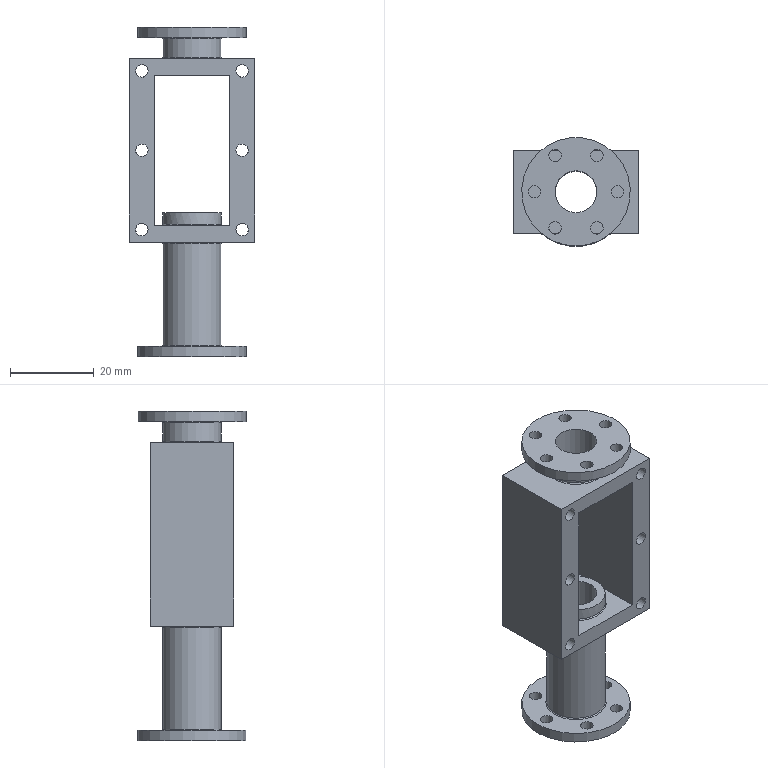Component | NX | WATER_TANK_CYL_BODY | 1 solid | 45 faces | volume 16504 mm3 | cylinder 25 | plane 15 | torus 5 | commonest cylinder face diameters 3 x18 14 x3 26 x2 10 x2